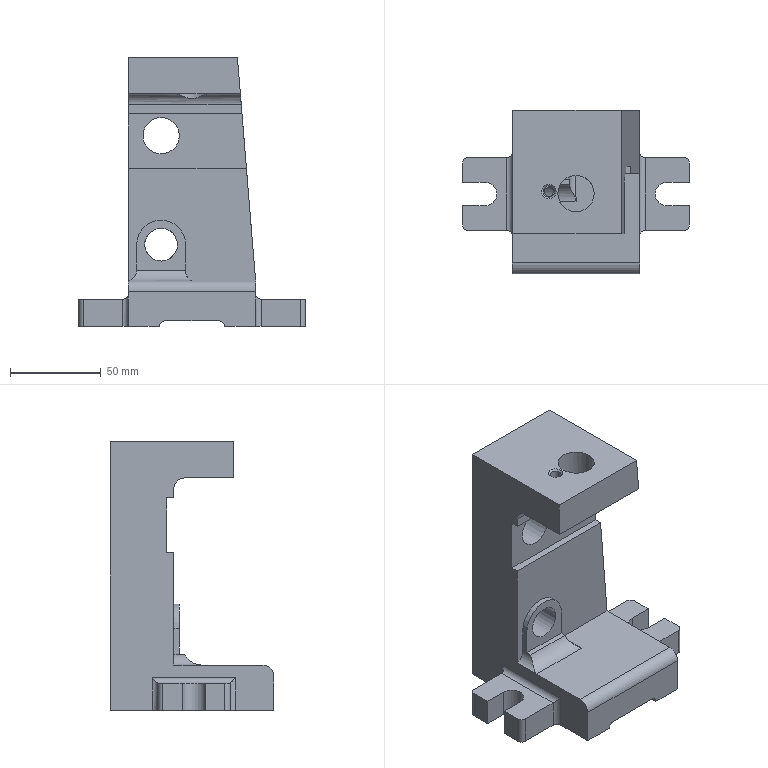Component | NX | STAND | 1 solid | 63 faces | volume 463949 mm3 | plane 36 | cylinder 25 | cone 2 | commonest cylinder face diameters 6 x12 12 x4 20 x3 13 x2 27 x1 18 x1 5 x1 6.1 x1